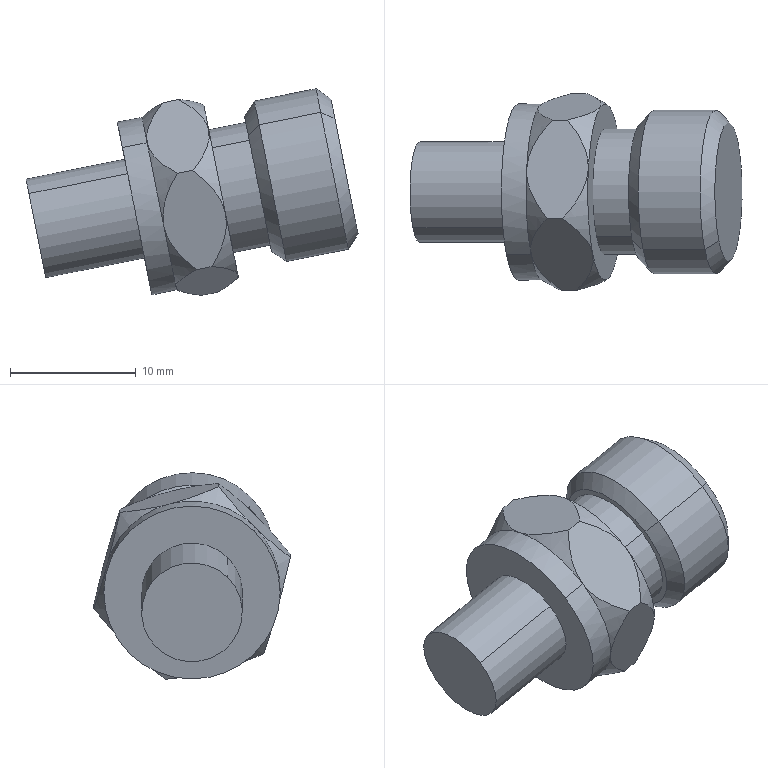Component | SolidWorks | 4-1 | 1 solid | 35 faces | volume 2667 mm3 | cone 16 | plane 11 | cylinder 8 | commonest cylinder face diameters 10 x2 13 x2 14 x2 8 x2